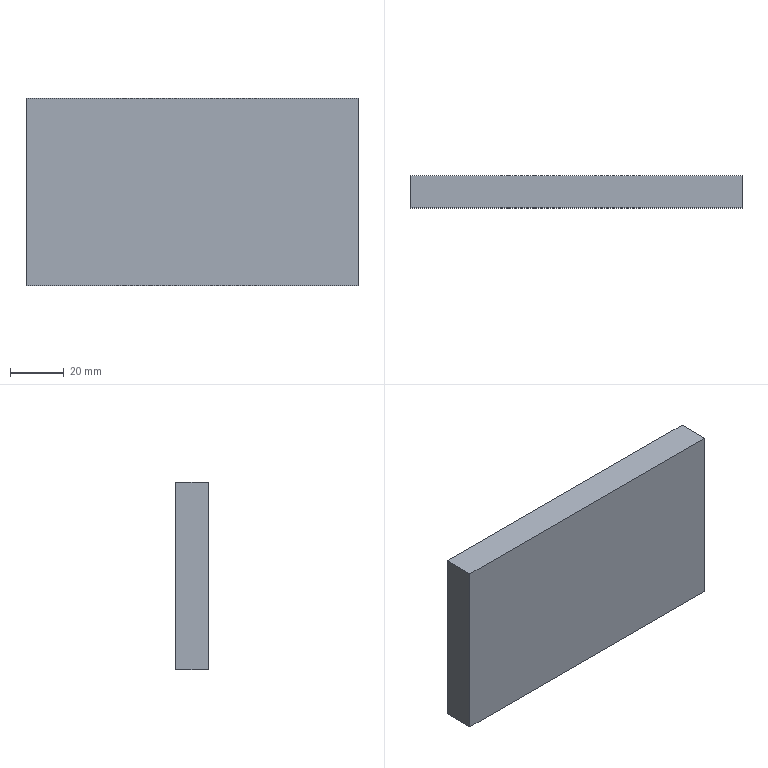Component | NX | CH3404_5-9_2 | 1 solid | 6 faces | box 124 x 12 x 70 mm | volume 104160 mm3 | plane 6
STEP:
#1=CARTESIAN_POINT('',(0.,0.,0.));
#2=DIRECTION('',(0.,0.,1.));
#3=DIRECTION('',(1.,0.,0.));
#4=AXIS2_PLACEMENT_3D('',#1,#2,#3);
#5=CARTESIAN_POINT('',(155.,80.,1670.));
#6=VERTEX_POINT('',#5);
#7=CARTESIAN_POINT('',(155.,80.,1600.));
#8=VERTEX_POINT('',#7);
#9=CARTESIAN_POINT('',(155.,80.,1670.));
#10=DIRECTION('',(0.,0.,-1.));
#11=VECTOR('',#10,1.);
#12=LINE('',#9,#11);
#13=CARTESIAN_POINT('',(155.,68.,1670.));
#14=DIRECTION('',(1.,0.,0.));
#15=DIRECTION('',(0.,0.,1.));
#16=AXIS2_PLACEMENT_3D('',#13,#14,#15);
#17=PLANE('',#16);
#18=CARTESIAN_POINT('',(0.,-12.));
#19=DIRECTION('',(-1.,0.));
#20=VECTOR('',#19,1.);
#21=LINE('',#18,#20);
#22=(GEOMETRIC_REPRESENTATION_CONTEXT(2)PARAMETRIC_REPRESENTATION_CONTEXT()REPRESENTATION_CONTEXT('',''));
#23=DEFINITIONAL_REPRESENTATION('',(#21),#22);
#24=PCURVE('',#17,#23);
#25=CARTESIAN_POINT('',(217.,80.,1635.));
#26=DIRECTION('',(0.,-1.,0.));
#27=DIRECTION('',(0.,0.,-1.));
#28=AXIS2_PLACEMENT_3D('',#25,#26,#27);
#29=PLANE('',#28);
#30=CARTESIAN_POINT('',(-35.,-62.));
#31=DIRECTION('',(1.,0.));
#32=VECTOR('',#31,1.);
#33=LINE('',#30,#32);
#34=(GEOMETRIC_REPRESENTATION_CONTEXT(2)PARAMETRIC_REPRESENTATION_CONTEXT()REPRESENTATION_CONTEXT('',''));
#35=DEFINITIONAL_REPRESENTATION('',(#33),#34);
#36=PCURVE('',#29,#35);
#37=SURFACE_CURVE('',#12,(#24,#36),.PCURVE_S1.);
#38=EDGE_CURVE('',#6,#8,#37,.T.);
#39=ORIENTED_EDGE('',*,*,#38,.T.);
#40=CARTESIAN_POINT('',(155.,68.,1600.));
#41=VERTEX_POINT('',#40);
#42=CARTESIAN_POINT('',(155.,68.,1600.));
#43=DIRECTION('',(0.,1.,0.));
#44=VECTOR('',#43,1.);
#45=LINE('',#42,#44);
#46=CARTESIAN_POINT('',(-70.,0.));
#47=DIRECTION('',(0.,-1.));
#48=VECTOR('',#47,1.);
#49=LINE('',#46,#48);
#50=(GEOMETRIC_REPRESENTATION_CONTEXT(2)PARAMETRIC_REPRESENTATION_CONTEXT()REPRESENTATION_CONTEXT('',''));
#51=DEFINITIONAL_REPRESENTATION('',(#49),#50);
#52=PCURVE('',#17,#51);
#53=CARTESIAN_POINT('',(155.,68.,1600.));
#54=DIRECTION('',(0.,0.,1.));
#55=DIRECTION('',(0.,-1.,0.));
#56=AXIS2_PLACEMENT_3D('',#53,#54,#55);
#57=PLANE('',#56);
#58=CARTESIAN_POINT('',(0.,0.));
#59=DIRECTION('',(-1.,0.));
#60=VECTOR('',#59,1.);
#61=LINE('',#58,#60);
#62=(GEOMETRIC_REPRESENTATION_CONTEXT(2)PARAMETRIC_REPRESENTATION_CONTEXT()REPRESENTATION_CONTEXT('',''));
#63=DEFINITIONAL_REPRESENTATION('',(#61),#62);
#64=PCURVE('',#57,#63);
#65=SURFACE_CURVE('',#45,(#52,#64),.PCURVE_S1.);
#66=EDGE_CURVE('',#41,#8,#65,.T.);
#67=ORIENTED_EDGE('',*,*,#66,.F.);
#68=CARTESIAN_POINT('',(155.,68.,1670.));
#69=VERTEX_POINT('',#68);
#70=CARTESIAN_POINT('',(155.,68.,1670.));
#71=DIRECTION('',(0.,0.,-1.));
#72=VECTOR('',#71,1.);
#73=LINE('',#70,#72);
#74=CARTESIAN_POINT('',(0.,0.));
#75=DIRECTION('',(-1.,0.));
#76=VECTOR('',#75,1.);
#77=LINE('',#74,#76);
#78=(GEOMETRIC_REPRESENTATION_CONTEXT(2)PARAMETRIC_REPRESENTATION_CONTEXT()REPRESENTATION_CONTEXT('',''));
#79=DEFINITIONAL_REPRESENTATION('',(#77),#78);
#80=PCURVE('',#17,#79);
#81=CARTESIAN_POINT('',(217.,68.,1635.));
#82=DIRECTION('',(0.,-1.,0.));
#83=DIRECTION('',(0.,0.,-1.));
#84=AXIS2_PLACEMENT_3D('',#81,#82,#83);
#85=PLANE('',#84);
#86=CARTESIAN_POINT('',(-35.,-62.));
#87=DIRECTION('',(1.,0.));
#88=VECTOR('',#87,1.);
#89=LINE('',#86,#88);
#90=(GEOMETRIC_REPRESENTATION_CONTEXT(2)PARAMETRIC_REPRESENTATION_CONTEXT()REPRESENTATION_CONTEXT('',''));
#91=DEFINITIONAL_REPRESENTATION('',(#89),#90);
#92=PCURVE('',#85,#91);
#93=SURFACE_CURVE('',#73,(#80,#92),.PCURVE_S1.);
#94=EDGE_CURVE('',#69,#41,#93,.T.);
#95=ORIENTED_EDGE('',*,*,#94,.F.);
#96=CARTESIAN_POINT('',(155.,68.,1670.));
#97=DIRECTION('',(0.,1.,0.));
#98=VECTOR('',#97,1.);
#99=LINE('',#96,#98);
#100=CARTESIAN_POINT('',(0.,0.));
#101=DIRECTION('',(0.,-1.));
#102=VECTOR('',#101,1.);
#103=LINE('',#100,#102);
#104=(GEOMETRIC_REPRESENTATION_CONTEXT(2)PARAMETRIC_REPRESENTATION_CONTEXT()REPRESENTATION_CONTEXT('',''));
#105=DEFINITIONAL_REPRESENTATION('',(#103),#104);
#106=PCURVE('',#17,#105);
#107=CARTESIAN_POINT('',(279.,68.,1670.));
#108=DIRECTION('',(0.,0.,-1.));
#109=DIRECTION('',(0.,1.,0.));
#110=AXIS2_PLACEMENT_3D('',#107,#108,#109);
#111=PLANE('',#110);
#112=CARTESIAN_POINT('',(0.,-124.));
#113=DIRECTION('',(1.,0.));
#114=VECTOR('',#113,1.);
#115=LINE('',#112,#114);
#116=(GEOMETRIC_REPRESENTATION_CONTEXT(2)PARAMETRIC_REPRESENTATION_CONTEXT()REPRESENTATION_CONTEXT('',''));
#117=DEFINITIONAL_REPRESENTATION('',(#115),#116);
#118=PCURVE('',#111,#117);
#119=SURFACE_CURVE('',#99,(#106,#118),.PCURVE_S1.);
#120=EDGE_CURVE('',#69,#6,#119,.T.);
#121=ORIENTED_EDGE('',*,*,#120,.T.);
#122=EDGE_LOOP('',(#39,#67,#95,#121));
#123=FACE_BOUND('',#122,.T.);
#124=ADVANCED_FACE('',(#123),#17,.F.);
#125=CARTESIAN_POINT('',(279.,80.,1600.));
#126=VERTEX_POINT('',#125);
#127=CARTESIAN_POINT('',(155.,80.,1600.));
#128=DIRECTION('',(1.,0.,0.));
#129=VECTOR('',#128,1.);
#130=LINE('',#127,#129);
#131=CARTESIAN_POINT('',(-12.,0.));
#132=DIRECTION('',(0.,1.));
#133=VECTOR('',#132,1.);
#134=LINE('',#131,#133);
#135=(GEOMETRIC_REPRESENTATION_CONTEXT(2)PARAMETRIC_REPRESENTATION_CONTEXT()REPRESENTATION_CONTEXT('',''));
#136=DEFINITIONAL_REPRESENTATION('',(#134),#135);
#137=PCURVE('',#57,#136);
#138=CARTESIAN_POINT('',(35.,-62.));
#139=DIRECTION('',(0.,1.));
#140=VECTOR('',#139,1.);
#141=LINE('',#138,#140);
#142=(GEOMETRIC_REPRESENTATION_CONTEXT(2)PARAMETRIC_REPRESENTATION_CONTEXT()REPRESENTATION_CONTEXT('',''));
#143=DEFINITIONAL_REPRESENTATION('',(#141),#142);
#144=PCURVE('',#29,#143);
#145=SURFACE_CURVE('',#130,(#137,#144),.PCURVE_S1.);
#146=EDGE_CURVE('',#8,#126,#145,.T.);
#147=ORIENTED_EDGE('',*,*,#146,.T.);
#148=CARTESIAN_POINT('',(279.,68.,1600.));
#149=VERTEX_POINT('',#148);
#150=CARTESIAN_POINT('',(279.,68.,1600.));
#151=DIRECTION('',(0.,1.,0.));
#152=VECTOR('',#151,1.);
#153=LINE('',#150,#152);
#154=CARTESIAN_POINT('',(0.,124.));
#155=DIRECTION('',(-1.,0.));
#156=VECTOR('',#155,1.);
#157=LINE('',#154,#156);
#158=(GEOMETRIC_REPRESENTATION_CONTEXT(2)PARAMETRIC_REPRESENTATION_CONTEXT()REPRESENTATION_CONTEXT('',''));
#159=DEFINITIONAL_REPRESENTATION('',(#157),#158);
#160=PCURVE('',#57,#159);
#161=CARTESIAN_POINT('',(279.,68.,1600.));
#162=DIRECTION('',(-1.,0.,0.));
#163=DIRECTION('',(0.,0.,-1.));
#164=AXIS2_PLACEMENT_3D('',#161,#162,#163);
#165=PLANE('',#164);
#166=CARTESIAN_POINT('',(0.,0.));
#167=DIRECTION('',(0.,-1.));
#168=VECTOR('',#167,1.);
#169=LINE('',#166,#168);
#170=(GEOMETRIC_REPRESENTATION_CONTEXT(2)PARAMETRIC_REPRESENTATION_CONTEXT()REPRESENTATION_CONTEXT('',''));
#171=DEFINITIONAL_REPRESENTATION('',(#169),#170);
#172=PCURVE('',#165,#171);
#173=SURFACE_CURVE('',#153,(#160,#172),.PCURVE_S1.);
#174=EDGE_CURVE('',#149,#126,#173,.T.);
#175=ORIENTED_EDGE('',*,*,#174,.F.);
#176=CARTESIAN_POINT('',(155.,68.,1600.));
#177=DIRECTION('',(1.,0.,0.));
#178=VECTOR('',#177,1.);
#179=LINE('',#176,#178);
#180=CARTESIAN_POINT('',(0.,0.));
#181=DIRECTION('',(0.,1.));
#182=VECTOR('',#181,1.);
#183=LINE('',#180,#182);
#184=(GEOMETRIC_REPRESENTATION_CONTEXT(2)PARAMETRIC_REPRESENTATION_CONTEXT()REPRESENTATION_CONTEXT('',''));
#185=DEFINITIONAL_REPRESENTATION('',(#183),#184);
#186=PCURVE('',#57,#185);
#187=CARTESIAN_POINT('',(35.,-62.));
#188=DIRECTION('',(0.,1.));
#189=VECTOR('',#188,1.);
#190=LINE('',#187,#189);
#191=(GEOMETRIC_REPRESENTATION_CONTEXT(2)PARAMETRIC_REPRESENTATION_CONTEXT()REPRESENTATION_CONTEXT('',''));
#192=DEFINITIONAL_REPRESENTATION('',(#190),#191);
#193=PCURVE('',#85,#192);
#194=SURFACE_CURVE('',#179,(#186,#193),.PCURVE_S1.);
#195=EDGE_CURVE('',#41,#149,#194,.T.);
#196=ORIENTED_EDGE('',*,*,#195,.F.);
#197=ORIENTED_EDGE('',*,*,#66,.T.);
#198=EDGE_LOOP('',(#147,#175,#196,#197));
#199=FACE_BOUND('',#198,.T.);
#200=ADVANCED_FACE('',(#199),#57,.F.);
#201=CARTESIAN_POINT('',(279.,80.,1670.));
#202=VERTEX_POINT('',#201);
#203=CARTESIAN_POINT('',(279.,80.,1600.));
#204=DIRECTION('',(0.,0.,1.));
#205=VECTOR('',#204,1.);
#206=LINE('',#203,#205);
#207=CARTESIAN_POINT('',(0.,-12.));
#208=DIRECTION('',(-1.,0.));
#209=VECTOR('',#208,1.);
#210=LINE('',#207,#209);
#211=(GEOMETRIC_REPRESENTATION_CONTEXT(2)PARAMETRIC_REPRESENTATION_CONTEXT()REPRESENTATION_CONTEXT('',''));
#212=DEFINITIONAL_REPRESENTATION('',(#210),#211);
#213=PCURVE('',#165,#212);
#214=CARTESIAN_POINT('',(35.,62.));
#215=DIRECTION('',(-1.,0.));
#216=VECTOR('',#215,1.);
#217=LINE('',#214,#216);
#218=(GEOMETRIC_REPRESENTATION_CONTEXT(2)PARAMETRIC_REPRESENTATION_CONTEXT()REPRESENTATION_CONTEXT('',''));
#219=DEFINITIONAL_REPRESENTATION('',(#217),#218);
#220=PCURVE('',#29,#219);
#221=SURFACE_CURVE('',#206,(#213,#220),.PCURVE_S1.);
#222=EDGE_CURVE('',#126,#202,#221,.T.);
#223=ORIENTED_EDGE('',*,*,#222,.T.);
#224=CARTESIAN_POINT('',(279.,68.,1670.));
#225=VERTEX_POINT('',#224);
#226=CARTESIAN_POINT('',(279.,68.,1670.));
#227=DIRECTION('',(0.,1.,0.));
#228=VECTOR('',#227,1.);
#229=LINE('',#226,#228);
#230=CARTESIAN_POINT('',(-70.,0.));
#231=DIRECTION('',(0.,-1.));
#232=VECTOR('',#231,1.);
#233=LINE('',#230,#232);
#234=(GEOMETRIC_REPRESENTATION_CONTEXT(2)PARAMETRIC_REPRESENTATION_CONTEXT()REPRESENTATION_CONTEXT('',''));
#235=DEFINITIONAL_REPRESENTATION('',(#233),#234);
#236=PCURVE('',#165,#235);
#237=CARTESIAN_POINT('',(0.,0.));
#238=DIRECTION('',(1.,0.));
#239=VECTOR('',#238,1.);
#240=LINE('',#237,#239);
#241=(GEOMETRIC_REPRESENTATION_CONTEXT(2)PARAMETRIC_REPRESENTATION_CONTEXT()REPRESENTATION_CONTEXT('',''));
#242=DEFINITIONAL_REPRESENTATION('',(#240),#241);
#243=PCURVE('',#111,#242);
#244=SURFACE_CURVE('',#229,(#236,#243),.PCURVE_S1.);
#245=EDGE_CURVE('',#225,#202,#244,.T.);
#246=ORIENTED_EDGE('',*,*,#245,.F.);
#247=CARTESIAN_POINT('',(279.,68.,1600.));
#248=DIRECTION('',(0.,0.,1.));
#249=VECTOR('',#248,1.);
#250=LINE('',#247,#249);
#251=CARTESIAN_POINT('',(0.,0.));
#252=DIRECTION('',(-1.,0.));
#253=VECTOR('',#252,1.);
#254=LINE('',#251,#253);
#255=(GEOMETRIC_REPRESENTATION_CONTEXT(2)PARAMETRIC_REPRESENTATION_CONTEXT()REPRESENTATION_CONTEXT('',''));
#256=DEFINITIONAL_REPRESENTATION('',(#254),#255);
#257=PCURVE('',#165,#256);
#258=CARTESIAN_POINT('',(35.,62.));
#259=DIRECTION('',(-1.,0.));
#260=VECTOR('',#259,1.);
#261=LINE('',#258,#260);
#262=(GEOMETRIC_REPRESENTATION_CONTEXT(2)PARAMETRIC_REPRESENTATION_CONTEXT()REPRESENTATION_CONTEXT('',''));
#263=DEFINITIONAL_REPRESENTATION('',(#261),#262);
#264=PCURVE('',#85,#263);
#265=SURFACE_CURVE('',#250,(#257,#264),.PCURVE_S1.);
#266=EDGE_CURVE('',#149,#225,#265,.T.);
#267=ORIENTED_EDGE('',*,*,#266,.F.);
#268=ORIENTED_EDGE('',*,*,#174,.T.);
#269=EDGE_LOOP('',(#223,#246,#267,#268));
#270=FACE_BOUND('',#269,.T.);
#271=ADVANCED_FACE('',(#270),#165,.F.);
#272=CARTESIAN_POINT('',(279.,80.,1670.));
#273=DIRECTION('',(-1.,0.,0.));
#274=VECTOR('',#273,1.);
#275=LINE('',#272,#274);
#276=CARTESIAN_POINT('',(12.,0.));
#277=DIRECTION('',(0.,-1.));
#278=VECTOR('',#277,1.);
#279=LINE('',#276,#278);
#280=(GEOMETRIC_REPRESENTATION_CONTEXT(2)PARAMETRIC_REPRESENTATION_CONTEXT()REPRESENTATION_CONTEXT('',''));
#281=DEFINITIONAL_REPRESENTATION('',(#279),#280);
#282=PCURVE('',#111,#281);
#283=CARTESIAN_POINT('',(-35.,62.));
#284=DIRECTION('',(0.,-1.));
#285=VECTOR('',#284,1.);
#286=LINE('',#283,#285);
#287=(GEOMETRIC_REPRESENTATION_CONTEXT(2)PARAMETRIC_REPRESENTATION_CONTEXT()REPRESENTATION_CONTEXT('',''));
#288=DEFINITIONAL_REPRESENTATION('',(#286),#287);
#289=PCURVE('',#29,#288);
#290=SURFACE_CURVE('',#275,(#282,#289),.PCURVE_S1.);
#291=EDGE_CURVE('',#202,#6,#290,.T.);
#292=ORIENTED_EDGE('',*,*,#291,.T.);
#293=ORIENTED_EDGE('',*,*,#120,.F.);
#294=CARTESIAN_POINT('',(279.,68.,1670.));
#295=DIRECTION('',(-1.,0.,0.));
#296=VECTOR('',#295,1.);
#297=LINE('',#294,#296);
#298=CARTESIAN_POINT('',(0.,0.));
#299=DIRECTION('',(0.,-1.));
#300=VECTOR('',#299,1.);
#301=LINE('',#298,#300);
#302=(GEOMETRIC_REPRESENTATION_CONTEXT(2)PARAMETRIC_REPRESENTATION_CONTEXT()REPRESENTATION_CONTEXT('',''));
#303=DEFINITIONAL_REPRESENTATION('',(#301),#302);
#304=PCURVE('',#111,#303);
#305=CARTESIAN_POINT('',(-35.,62.));
#306=DIRECTION('',(0.,-1.));
#307=VECTOR('',#306,1.);
#308=LINE('',#305,#307);
#309=(GEOMETRIC_REPRESENTATION_CONTEXT(2)PARAMETRIC_REPRESENTATION_CONTEXT()REPRESENTATION_CONTEXT('',''));
#310=DEFINITIONAL_REPRESENTATION('',(#308),#309);
#311=PCURVE('',#85,#310);
#312=SURFACE_CURVE('',#297,(#304,#311),.PCURVE_S1.);
#313=EDGE_CURVE('',#225,#69,#312,.T.);
#314=ORIENTED_EDGE('',*,*,#313,.F.);
#315=ORIENTED_EDGE('',*,*,#245,.T.);
#316=EDGE_LOOP('',(#292,#293,#314,#315));
#317=FACE_BOUND('',#316,.T.);
#318=ADVANCED_FACE('',(#317),#111,.F.);
#319=ORIENTED_EDGE('',*,*,#94,.T.);
#320=ORIENTED_EDGE('',*,*,#195,.T.);
#321=ORIENTED_EDGE('',*,*,#266,.T.);
#322=ORIENTED_EDGE('',*,*,#313,.T.);
#323=EDGE_LOOP('',(#319,#320,#321,#322));
#324=FACE_BOUND('',#323,.T.);
#325=ADVANCED_FACE('',(#324),#85,.T.);
#326=ORIENTED_EDGE('',*,*,#38,.F.);
#327=ORIENTED_EDGE('',*,*,#291,.F.);
#328=ORIENTED_EDGE('',*,*,#222,.F.);
#329=ORIENTED_EDGE('',*,*,#146,.F.);
#330=EDGE_LOOP('',(#326,#327,#328,#329));
#331=FACE_BOUND('',#330,.T.);
#332=ADVANCED_FACE('',(#331),#29,.F.);
#333=CLOSED_SHELL('',(#124,#200,#271,#318,#325,#332));
#334=MANIFOLD_SOLID_BREP('',#333);
#335=(LENGTH_UNIT()NAMED_UNIT(*)SI_UNIT(.MILLI.,.METRE.));
#336=UNCERTAINTY_MEASURE_WITH_UNIT(LENGTH_MEASURE(0.0000001),#335,'','');
#337=(NAMED_UNIT(*)PLANE_ANGLE_UNIT()SI_UNIT($,.RADIAN.));
#338=(NAMED_UNIT(*)SI_UNIT($,.STERADIAN.)SOLID_ANGLE_UNIT());
#339=(GEOMETRIC_REPRESENTATION_CONTEXT(3)GLOBAL_UNCERTAINTY_ASSIGNED_CONTEXT((#336))GLOBAL_UNIT_ASSIGNED_CONTEXT((#335,#337,#338))REPRESENTATION_CONTEXT('',''));
#340=ADVANCED_BREP_SHAPE_REPRESENTATION('',(#4,#334),#339);